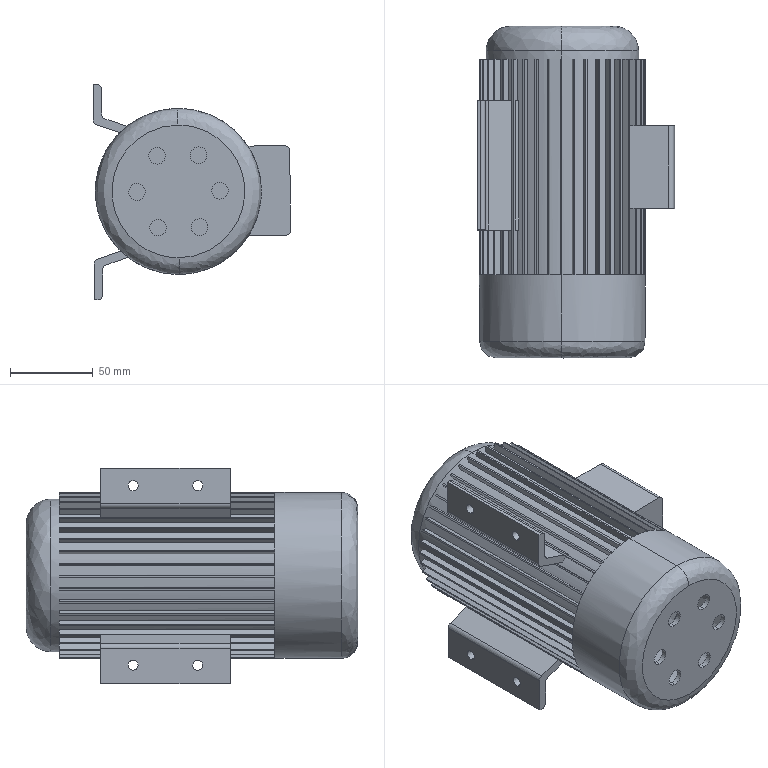Component | SolidWorks | LX-TSJ-05-1 | 1 solid | 306 faces | volume 319328 mm3 | plane 252 | cylinder 46 | spline 8 | commonest cylinder face diameters 6 x16 10 x12 92 x10 86 x2 94 x2 20 x2 100 x2